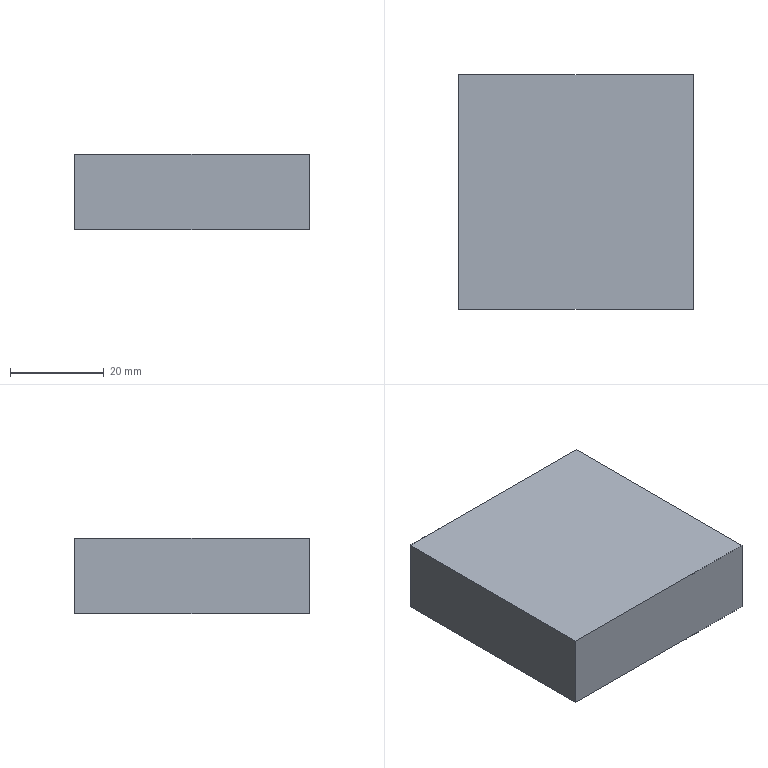Component | SolidWorks | TractionSmallCylinderSeat-1 | 1 solid | 14 faces | box 50 x 50 x 16 mm | volume 36700 mm3 | plane 6 | cylinder 4 | cone 4 | commonest cylinder face diameters 8.8 x4
build123d program:
from build123d import *

# Parameters (mm, degrees)
SKETCH1_W                   = 50
SKETCH1_H                   = 50
EXTRUDE1_DEPTH              = 16
M10X1_25_TAPPED_HOLE1_D     = 8.8
M10X1_25_TAPPED_HOLE1_DEPTH = 26.25
M10X1_25_TAPPED_HOLE1_TIP   = 2.644


with BuildPart() as part:
    # Sketch1 → Extrude1 (new body)
    with BuildSketch(Plane.XY):
        with Locations((-0.4613, -9.068)):
            Rectangle(SKETCH1_W, SKETCH1_H)
    extrude(amount=EXTRUDE1_DEPTH)

    # M10x1.25 Tapped Hole1
    with Locations(Plane(origin=(0, 15.932, 0), x_dir=(-1, 0, 0), z_dir=(0, 1, 0))):
        with Locations((17.961, 8), (-17.039, 8)):
            Hole(M10X1_25_TAPPED_HOLE1_D / 2, depth=M10X1_25_TAPPED_HOLE1_DEPTH)
            with Locations((0, 0, -(M10X1_25_TAPPED_HOLE1_DEPTH + M10X1_25_TAPPED_HOLE1_TIP / 2))):  # 118° drill point
                Cone(0, M10X1_25_TAPPED_HOLE1_D / 2, M10X1_25_TAPPED_HOLE1_TIP, mode=Mode.SUBTRACT)


solid = part.part

# Placed as in the assembly
solid = solid.moved(Location((250.678, 472.052, 76.106), (0, 0, 0)))
STEP:
#1=COLOUR_RGB('',0.7922,0.8196,0.9333);
#2=FILL_AREA_STYLE_COLOUR('',#1);
#3=FILL_AREA_STYLE('',(#2));
#4=SURFACE_STYLE_FILL_AREA(#3);
#5=SURFACE_SIDE_STYLE('',(#4));
#6=SURFACE_STYLE_USAGE(.BOTH.,#5);
#7=PRESENTATION_STYLE_ASSIGNMENT((#6));
#8=CARTESIAN_POINT('',(9.162,18.178,3.138));
#9=VERTEX_POINT('',#8);
#10=CARTESIAN_POINT('',(9.162,18.178,3.484));
#11=VERTEX_POINT('',#10);
#12=CARTESIAN_POINT('',(9.162,18.178,3.311));
#13=DIRECTION('',(0.,1.,0.));
#14=DIRECTION('',(0.,0.,1.));
#15=AXIS2_PLACEMENT_3D('',#12,#13,#14);
#16=CIRCLE('',#15,0.1732);
#17=EDGE_CURVE('',#9,#11,#16,.T.);
#18=ORIENTED_EDGE('',*,*,#17,.F.);
#19=CARTESIAN_POINT('',(9.162,19.212,3.138));
#20=VERTEX_POINT('',#19);
#21=CARTESIAN_POINT('',(9.162,19.212,3.138));
#22=DIRECTION('',(0.,1.,0.));
#23=VECTOR('',#22,39.37);
#24=LINE('',#21,#23);
#25=EDGE_CURVE('',#9,#20,#24,.T.);
#26=ORIENTED_EDGE('',*,*,#25,.T.);
#27=CARTESIAN_POINT('',(9.162,19.212,3.484));
#28=VERTEX_POINT('',#27);
#29=CARTESIAN_POINT('',(9.162,19.212,3.311));
#30=DIRECTION('',(0.,1.,0.));
#31=DIRECTION('',(0.,0.,1.));
#32=AXIS2_PLACEMENT_3D('',#29,#30,#31);
#33=CIRCLE('',#32,0.1732);
#34=EDGE_CURVE('',#20,#28,#33,.T.);
#35=ORIENTED_EDGE('',*,*,#34,.T.);
#36=CARTESIAN_POINT('',(9.162,19.212,3.484));
#37=DIRECTION('',(0.,1.,0.));
#38=VECTOR('',#37,39.37);
#39=LINE('',#36,#38);
#40=EDGE_CURVE('',#11,#28,#39,.T.);
#41=ORIENTED_EDGE('',*,*,#40,.F.);
#42=EDGE_LOOP('',(#18,#26,#35,#41));
#43=FACE_OUTER_BOUND('',#42,.T.);
#44=CARTESIAN_POINT('',(9.162,19.212,3.311));
#45=DIRECTION('',(0.,1.,0.));
#46=DIRECTION('',(0.,0.,1.));
#47=AXIS2_PLACEMENT_3D('',#44,#45,#46);
#48=CYLINDRICAL_SURFACE('',#47,0.1732);
#49=ADVANCED_FACE('',(#43),#48,.F.);
#50=CARTESIAN_POINT('',(9.162,18.074,3.311));
#51=VERTEX_POINT('',#50);
#52=CARTESIAN_POINT('',(9.162,18.178,3.484));
#53=DIRECTION('',(0.,0.515,0.8572));
#54=VECTOR('',#53,39.37);
#55=LINE('',#52,#54);
#56=EDGE_CURVE('',#51,#11,#55,.T.);
#57=ORIENTED_EDGE('',*,*,#56,.F.);
#58=CARTESIAN_POINT('',(9.162,18.178,3.138));
#59=DIRECTION('',(0.,0.515,-0.8572));
#60=VECTOR('',#59,39.37);
#61=LINE('',#58,#60);
#62=EDGE_CURVE('',#51,#9,#61,.T.);
#63=ORIENTED_EDGE('',*,*,#62,.T.);
#64=ORIENTED_EDGE('',*,*,#17,.T.);
#65=EDGE_LOOP('',(#57,#63,#64));
#66=FACE_OUTER_BOUND('',#65,.T.);
#67=CARTESIAN_POINT('',(9.162,18.178,3.311));
#68=DIRECTION('',(0.,1.,0.));
#69=DIRECTION('',(0.,0.,1.));
#70=AXIS2_PLACEMENT_3D('',#67,#68,#69);
#71=CONICAL_SURFACE('',#70,0.1732,1.03);
#72=ADVANCED_FACE('',(#66),#71,.F.);
#73=CARTESIAN_POINT('',(10.54,18.178,3.138));
#74=VERTEX_POINT('',#73);
#75=CARTESIAN_POINT('',(10.54,18.178,3.484));
#76=VERTEX_POINT('',#75);
#77=CARTESIAN_POINT('',(10.54,18.178,3.311));
#78=DIRECTION('',(0.,1.,0.));
#79=DIRECTION('',(0.,0.,1.));
#80=AXIS2_PLACEMENT_3D('',#77,#78,#79);
#81=CIRCLE('',#80,0.1732);
#82=EDGE_CURVE('',#74,#76,#81,.T.);
#83=ORIENTED_EDGE('',*,*,#82,.F.);
#84=CARTESIAN_POINT('',(10.54,19.212,3.138));
#85=VERTEX_POINT('',#84);
#86=CARTESIAN_POINT('',(10.54,19.212,3.138));
#87=DIRECTION('',(0.,1.,0.));
#88=VECTOR('',#87,39.37);
#89=LINE('',#86,#88);
#90=EDGE_CURVE('',#74,#85,#89,.T.);
#91=ORIENTED_EDGE('',*,*,#90,.T.);
#92=CARTESIAN_POINT('',(10.54,19.212,3.484));
#93=VERTEX_POINT('',#92);
#94=CARTESIAN_POINT('',(10.54,19.212,3.311));
#95=DIRECTION('',(0.,1.,0.));
#96=DIRECTION('',(0.,0.,1.));
#97=AXIS2_PLACEMENT_3D('',#94,#95,#96);
#98=CIRCLE('',#97,0.1732);
#99=EDGE_CURVE('',#85,#93,#98,.T.);
#100=ORIENTED_EDGE('',*,*,#99,.T.);
#101=CARTESIAN_POINT('',(10.54,19.212,3.484));
#102=DIRECTION('',(0.,1.,0.));
#103=VECTOR('',#102,39.37);
#104=LINE('',#101,#103);
#105=EDGE_CURVE('',#76,#93,#104,.T.);
#106=ORIENTED_EDGE('',*,*,#105,.F.);
#107=EDGE_LOOP('',(#83,#91,#100,#106));
#108=FACE_OUTER_BOUND('',#107,.T.);
#109=CARTESIAN_POINT('',(10.54,19.212,3.311));
#110=DIRECTION('',(0.,1.,0.));
#111=DIRECTION('',(0.,0.,1.));
#112=AXIS2_PLACEMENT_3D('',#109,#110,#111);
#113=CYLINDRICAL_SURFACE('',#112,0.1732);
#114=ADVANCED_FACE('',(#108),#113,.F.);
#115=CARTESIAN_POINT('',(10.54,18.074,3.311));
#116=VERTEX_POINT('',#115);
#117=CARTESIAN_POINT('',(10.54,18.178,3.484));
#118=DIRECTION('',(0.,0.515,0.8572));
#119=VECTOR('',#118,39.37);
#120=LINE('',#117,#119);
#121=EDGE_CURVE('',#116,#76,#120,.T.);
#122=ORIENTED_EDGE('',*,*,#121,.F.);
#123=CARTESIAN_POINT('',(10.54,18.178,3.138));
#124=DIRECTION('',(0.,0.515,-0.8572));
#125=VECTOR('',#124,39.37);
#126=LINE('',#123,#125);
#127=EDGE_CURVE('',#116,#74,#126,.T.);
#128=ORIENTED_EDGE('',*,*,#127,.T.);
#129=ORIENTED_EDGE('',*,*,#82,.T.);
#130=EDGE_LOOP('',(#122,#128,#129));
#131=FACE_OUTER_BOUND('',#130,.T.);
#132=CARTESIAN_POINT('',(10.54,18.178,3.311));
#133=DIRECTION('',(0.,1.,0.));
#134=DIRECTION('',(0.,0.,1.));
#135=AXIS2_PLACEMENT_3D('',#132,#133,#134);
#136=CONICAL_SURFACE('',#135,0.1732,1.03);
#137=ADVANCED_FACE('',(#131),#136,.F.);
#138=CARTESIAN_POINT('',(8.867,19.212,2.996));
#139=VERTEX_POINT('',#138);
#140=CARTESIAN_POINT('',(8.867,17.243,2.996));
#141=VERTEX_POINT('',#140);
#142=CARTESIAN_POINT('',(8.867,19.212,2.996));
#143=DIRECTION('',(0.,-1.,0.));
#144=VECTOR('',#143,39.37);
#145=LINE('',#142,#144);
#146=EDGE_CURVE('',#139,#141,#145,.T.);
#147=ORIENTED_EDGE('',*,*,#146,.T.);
#148=CARTESIAN_POINT('',(8.867,17.243,3.626));
#149=VERTEX_POINT('',#148);
#150=CARTESIAN_POINT('',(8.867,17.243,3.626));
#151=DIRECTION('',(0.,0.,-1.));
#152=VECTOR('',#151,39.37);
#153=LINE('',#150,#152);
#154=EDGE_CURVE('',#149,#141,#153,.T.);
#155=ORIENTED_EDGE('',*,*,#154,.F.);
#156=CARTESIAN_POINT('',(8.867,19.212,3.626));
#157=VERTEX_POINT('',#156);
#158=CARTESIAN_POINT('',(8.867,19.212,3.626));
#159=DIRECTION('',(0.,-1.,0.));
#160=VECTOR('',#159,39.37);
#161=LINE('',#158,#160);
#162=EDGE_CURVE('',#157,#149,#161,.T.);
#163=ORIENTED_EDGE('',*,*,#162,.F.);
#164=CARTESIAN_POINT('',(8.867,19.212,3.626));
#165=DIRECTION('',(0.,0.,-1.));
#166=VECTOR('',#165,39.37);
#167=LINE('',#164,#166);
#168=EDGE_CURVE('',#157,#139,#167,.T.);
#169=ORIENTED_EDGE('',*,*,#168,.T.);
#170=EDGE_LOOP('',(#147,#155,#163,#169));
#171=FACE_OUTER_BOUND('',#170,.T.);
#172=CARTESIAN_POINT('',(8.867,19.212,3.626));
#173=DIRECTION('',(1.,0.,0.));
#174=DIRECTION('',(0.,0.,-1.));
#175=AXIS2_PLACEMENT_3D('',#172,#173,#174);
#176=PLANE('',#175);
#177=ADVANCED_FACE('',(#171),#176,.F.);
#178=CARTESIAN_POINT('',(10.835,17.243,2.996));
#179=VERTEX_POINT('',#178);
#180=CARTESIAN_POINT('',(8.867,17.243,2.996));
#181=DIRECTION('',(1.,0.,0.));
#182=VECTOR('',#181,39.37);
#183=LINE('',#180,#182);
#184=EDGE_CURVE('',#141,#179,#183,.T.);
#185=ORIENTED_EDGE('',*,*,#184,.T.);
#186=CARTESIAN_POINT('',(10.835,17.243,3.626));
#187=VERTEX_POINT('',#186);
#188=CARTESIAN_POINT('',(10.835,17.243,3.626));
#189=DIRECTION('',(0.,0.,-1.));
#190=VECTOR('',#189,39.37);
#191=LINE('',#188,#190);
#192=EDGE_CURVE('',#187,#179,#191,.T.);
#193=ORIENTED_EDGE('',*,*,#192,.F.);
#194=CARTESIAN_POINT('',(8.867,17.243,3.626));
#195=DIRECTION('',(1.,0.,0.));
#196=VECTOR('',#195,39.37);
#197=LINE('',#194,#196);
#198=EDGE_CURVE('',#149,#187,#197,.T.);
#199=ORIENTED_EDGE('',*,*,#198,.F.);
#200=ORIENTED_EDGE('',*,*,#154,.T.);
#201=EDGE_LOOP('',(#185,#193,#199,#200));
#202=FACE_OUTER_BOUND('',#201,.T.);
#203=CARTESIAN_POINT('',(8.867,17.243,3.626));
#204=DIRECTION('',(0.,1.,0.));
#205=DIRECTION('',(0.,0.,1.));
#206=AXIS2_PLACEMENT_3D('',#203,#204,#205);
#207=PLANE('',#206);
#208=ADVANCED_FACE('',(#202),#207,.F.);
#209=CARTESIAN_POINT('',(10.835,19.212,2.996));
#210=VERTEX_POINT('',#209);
#211=CARTESIAN_POINT('',(10.835,19.212,2.996));
#212=DIRECTION('',(-0.,1.,0.));
#213=VECTOR('',#212,39.37);
#214=LINE('',#211,#213);
#215=EDGE_CURVE('',#179,#210,#214,.T.);
#216=ORIENTED_EDGE('',*,*,#215,.T.);
#217=CARTESIAN_POINT('',(10.835,19.212,3.626));
#218=VERTEX_POINT('',#217);
#219=CARTESIAN_POINT('',(10.835,19.212,3.626));
#220=DIRECTION('',(0.,0.,-1.));
#221=VECTOR('',#220,39.37);
#222=LINE('',#219,#221);
#223=EDGE_CURVE('',#218,#210,#222,.T.);
#224=ORIENTED_EDGE('',*,*,#223,.F.);
#225=CARTESIAN_POINT('',(10.835,19.212,3.626));
#226=DIRECTION('',(-0.,1.,0.));
#227=VECTOR('',#226,39.37);
#228=LINE('',#225,#227);
#229=EDGE_CURVE('',#187,#218,#228,.T.);
#230=ORIENTED_EDGE('',*,*,#229,.F.);
#231=ORIENTED_EDGE('',*,*,#192,.T.);
#232=EDGE_LOOP('',(#216,#224,#230,#231));
#233=FACE_OUTER_BOUND('',#232,.T.);
#234=CARTESIAN_POINT('',(10.835,19.212,3.626));
#235=DIRECTION('',(-1.,-0.,0.));
#236=DIRECTION('',(0.,-1.,0.));
#237=AXIS2_PLACEMENT_3D('',#234,#235,#236);
#238=PLANE('',#237);
#239=ADVANCED_FACE('',(#233),#238,.F.);
#240=CARTESIAN_POINT('',(9.162,19.212,3.311));
#241=DIRECTION('',(0.,1.,0.));
#242=DIRECTION('',(0.,0.,1.));
#243=AXIS2_PLACEMENT_3D('',#240,#241,#242);
#244=CIRCLE('',#243,0.1732);
#245=EDGE_CURVE('',#28,#20,#244,.T.);
#246=ORIENTED_EDGE('',*,*,#245,.F.);
#247=ORIENTED_EDGE('',*,*,#34,.F.);
#248=EDGE_LOOP('',(#246,#247));
#249=FACE_BOUND('',#248,.T.);
#250=CARTESIAN_POINT('',(10.54,19.212,3.311));
#251=DIRECTION('',(0.,1.,0.));
#252=DIRECTION('',(0.,0.,1.));
#253=AXIS2_PLACEMENT_3D('',#250,#251,#252);
#254=CIRCLE('',#253,0.1732);
#255=EDGE_CURVE('',#93,#85,#254,.T.);
#256=ORIENTED_EDGE('',*,*,#255,.F.);
#257=ORIENTED_EDGE('',*,*,#99,.F.);
#258=EDGE_LOOP('',(#256,#257));
#259=FACE_BOUND('',#258,.T.);
#260=CARTESIAN_POINT('',(8.867,19.212,2.996));
#261=DIRECTION('',(-1.,0.,0.));
#262=VECTOR('',#261,39.37);
#263=LINE('',#260,#262);
#264=EDGE_CURVE('',#210,#139,#263,.T.);
#265=ORIENTED_EDGE('',*,*,#264,.T.);
#266=ORIENTED_EDGE('',*,*,#168,.F.);
#267=CARTESIAN_POINT('',(8.867,19.212,3.626));
#268=DIRECTION('',(-1.,0.,0.));
#269=VECTOR('',#268,39.37);
#270=LINE('',#267,#269);
#271=EDGE_CURVE('',#218,#157,#270,.T.);
#272=ORIENTED_EDGE('',*,*,#271,.F.);
#273=ORIENTED_EDGE('',*,*,#223,.T.);
#274=EDGE_LOOP('',(#265,#266,#272,#273));
#275=FACE_OUTER_BOUND('',#274,.T.);
#276=CARTESIAN_POINT('',(8.867,19.212,3.626));
#277=DIRECTION('',(0.,-1.,0.));
#278=DIRECTION('',(0.,0.,-1.));
#279=AXIS2_PLACEMENT_3D('',#276,#277,#278);
#280=PLANE('',#279);
#281=ADVANCED_FACE('',(#249,#259,#275),#280,.F.);
#282=ORIENTED_EDGE('',*,*,#162,.T.);
#283=ORIENTED_EDGE('',*,*,#198,.T.);
#284=ORIENTED_EDGE('',*,*,#229,.T.);
#285=ORIENTED_EDGE('',*,*,#271,.T.);
#286=EDGE_LOOP('',(#282,#283,#284,#285));
#287=FACE_OUTER_BOUND('',#286,.T.);
#288=CARTESIAN_POINT('',(8.867,17.243,3.626));
#289=DIRECTION('',(0.,0.,1.));
#290=DIRECTION('',(1.,0.,0.));
#291=AXIS2_PLACEMENT_3D('',#288,#289,#290);
#292=PLANE('',#291);
#293=ADVANCED_FACE('',(#287),#292,.T.);
#294=ORIENTED_EDGE('',*,*,#146,.F.);
#295=ORIENTED_EDGE('',*,*,#264,.F.);
#296=ORIENTED_EDGE('',*,*,#215,.F.);
#297=ORIENTED_EDGE('',*,*,#184,.F.);
#298=EDGE_LOOP('',(#294,#295,#296,#297));
#299=FACE_OUTER_BOUND('',#298,.T.);
#300=CARTESIAN_POINT('',(8.867,17.243,2.996));
#301=DIRECTION('',(0.,0.,1.));
#302=DIRECTION('',(1.,0.,0.));
#303=AXIS2_PLACEMENT_3D('',#300,#301,#302);
#304=PLANE('',#303);
#305=ADVANCED_FACE('',(#299),#304,.F.);
#306=ORIENTED_EDGE('',*,*,#127,.F.);
#307=ORIENTED_EDGE('',*,*,#121,.T.);
#308=CARTESIAN_POINT('',(10.54,18.178,3.311));
#309=DIRECTION('',(0.,1.,0.));
#310=DIRECTION('',(0.,0.,1.));
#311=AXIS2_PLACEMENT_3D('',#308,#309,#310);
#312=CIRCLE('',#311,0.1732);
#313=EDGE_CURVE('',#76,#74,#312,.T.);
#314=ORIENTED_EDGE('',*,*,#313,.T.);
#315=EDGE_LOOP('',(#306,#307,#314));
#316=FACE_OUTER_BOUND('',#315,.T.);
#317=CARTESIAN_POINT('',(10.54,18.178,3.311));
#318=DIRECTION('',(0.,1.,0.));
#319=DIRECTION('',(0.,0.,1.));
#320=AXIS2_PLACEMENT_3D('',#317,#318,#319);
#321=CONICAL_SURFACE('',#320,0.1732,1.03);
#322=ADVANCED_FACE('',(#316),#321,.F.);
#323=ORIENTED_EDGE('',*,*,#90,.F.);
#324=ORIENTED_EDGE('',*,*,#313,.F.);
#325=ORIENTED_EDGE('',*,*,#105,.T.);
#326=ORIENTED_EDGE('',*,*,#255,.T.);
#327=EDGE_LOOP('',(#323,#324,#325,#326));
#328=FACE_OUTER_BOUND('',#327,.T.);
#329=CARTESIAN_POINT('',(10.54,19.212,3.311));
#330=DIRECTION('',(0.,1.,0.));
#331=DIRECTION('',(0.,0.,1.));
#332=AXIS2_PLACEMENT_3D('',#329,#330,#331);
#333=CYLINDRICAL_SURFACE('',#332,0.1732);
#334=ADVANCED_FACE('',(#328),#333,.F.);
#335=ORIENTED_EDGE('',*,*,#62,.F.);
#336=ORIENTED_EDGE('',*,*,#56,.T.);
#337=CARTESIAN_POINT('',(9.162,18.178,3.311));
#338=DIRECTION('',(0.,1.,0.));
#339=DIRECTION('',(0.,0.,1.));
#340=AXIS2_PLACEMENT_3D('',#337,#338,#339);
#341=CIRCLE('',#340,0.1732);
#342=EDGE_CURVE('',#11,#9,#341,.T.);
#343=ORIENTED_EDGE('',*,*,#342,.T.);
#344=EDGE_LOOP('',(#335,#336,#343));
#345=FACE_OUTER_BOUND('',#344,.T.);
#346=CARTESIAN_POINT('',(9.162,18.178,3.311));
#347=DIRECTION('',(0.,1.,0.));
#348=DIRECTION('',(0.,0.,1.));
#349=AXIS2_PLACEMENT_3D('',#346,#347,#348);
#350=CONICAL_SURFACE('',#349,0.1732,1.03);
#351=ADVANCED_FACE('',(#345),#350,.F.);
#352=ORIENTED_EDGE('',*,*,#25,.F.);
#353=ORIENTED_EDGE('',*,*,#342,.F.);
#354=ORIENTED_EDGE('',*,*,#40,.T.);
#355=ORIENTED_EDGE('',*,*,#245,.T.);
#356=EDGE_LOOP('',(#352,#353,#354,#355));
#357=FACE_OUTER_BOUND('',#356,.T.);
#358=CARTESIAN_POINT('',(9.162,19.212,3.311));
#359=DIRECTION('',(0.,1.,0.));
#360=DIRECTION('',(0.,0.,1.));
#361=AXIS2_PLACEMENT_3D('',#358,#359,#360);
#362=CYLINDRICAL_SURFACE('',#361,0.1732);
#363=ADVANCED_FACE('',(#357),#362,.F.);
#364=CLOSED_SHELL('',(#49,#72,#114,#137,#177,#208,#239,#281,#293,#305,#322,#334,#351,#363));
#365=MANIFOLD_SOLID_BREP('',#364);
#366=STYLED_ITEM('',(#7),#365);
#367=PRESENTATION_LAYER_ASSIGNMENT('','',(#366));
#368=CARTESIAN_POINT('',(0.,0.,0.));
#369=DIRECTION('',(0.,0.,1.));
#370=DIRECTION('',(1.,0.,0.));
#371=AXIS2_PLACEMENT_3D('',#368,#369,#370);
#372=(LENGTH_UNIT()NAMED_UNIT(*)SI_UNIT($,.METRE.));
#373=LENGTH_MEASURE_WITH_UNIT(LENGTH_MEASURE(0.0254),#372);
#374=DIMENSIONAL_EXPONENTS(1.,0.,0.,0.,0.,0.,0.);
#375=(CONVERSION_BASED_UNIT('',#373)LENGTH_UNIT()NAMED_UNIT(#374));
#376=UNCERTAINTY_MEASURE_WITH_UNIT(LENGTH_MEASURE(0.00001),#375,'','');
#377=(NAMED_UNIT(*)PLANE_ANGLE_UNIT()SI_UNIT($,.RADIAN.));
#378=(NAMED_UNIT(*)SI_UNIT($,.STERADIAN.)SOLID_ANGLE_UNIT());
#379=(GEOMETRIC_REPRESENTATION_CONTEXT(3)GLOBAL_UNCERTAINTY_ASSIGNED_CONTEXT((#376))GLOBAL_UNIT_ASSIGNED_CONTEXT((#375,#377,#378))REPRESENTATION_CONTEXT('',''));
#380=ADVANCED_BREP_SHAPE_REPRESENTATION('',(#365,#371),#379);
#381=(LENGTH_UNIT()NAMED_UNIT(*)SI_UNIT($,.METRE.));
#382=LENGTH_MEASURE_WITH_UNIT(LENGTH_MEASURE(0.0254),#381);
#383=DIMENSIONAL_EXPONENTS(1.,0.,0.,0.,0.,0.,0.);
#384=(CONVERSION_BASED_UNIT('',#382)LENGTH_UNIT()NAMED_UNIT(#383));
#385=UNCERTAINTY_MEASURE_WITH_UNIT(LENGTH_MEASURE(0.00001),#384,'','');
#386=(NAMED_UNIT(*)PLANE_ANGLE_UNIT()SI_UNIT($,.RADIAN.));
#387=(NAMED_UNIT(*)SI_UNIT($,.STERADIAN.)SOLID_ANGLE_UNIT());
#388=(GEOMETRIC_REPRESENTATION_CONTEXT(3)GLOBAL_UNCERTAINTY_ASSIGNED_CONTEXT((#385))GLOBAL_UNIT_ASSIGNED_CONTEXT((#384,#386,#387))REPRESENTATION_CONTEXT('',''));
#389=MECHANICAL_DESIGN_GEOMETRIC_PRESENTATION_REPRESENTATION('',(#366),#388);